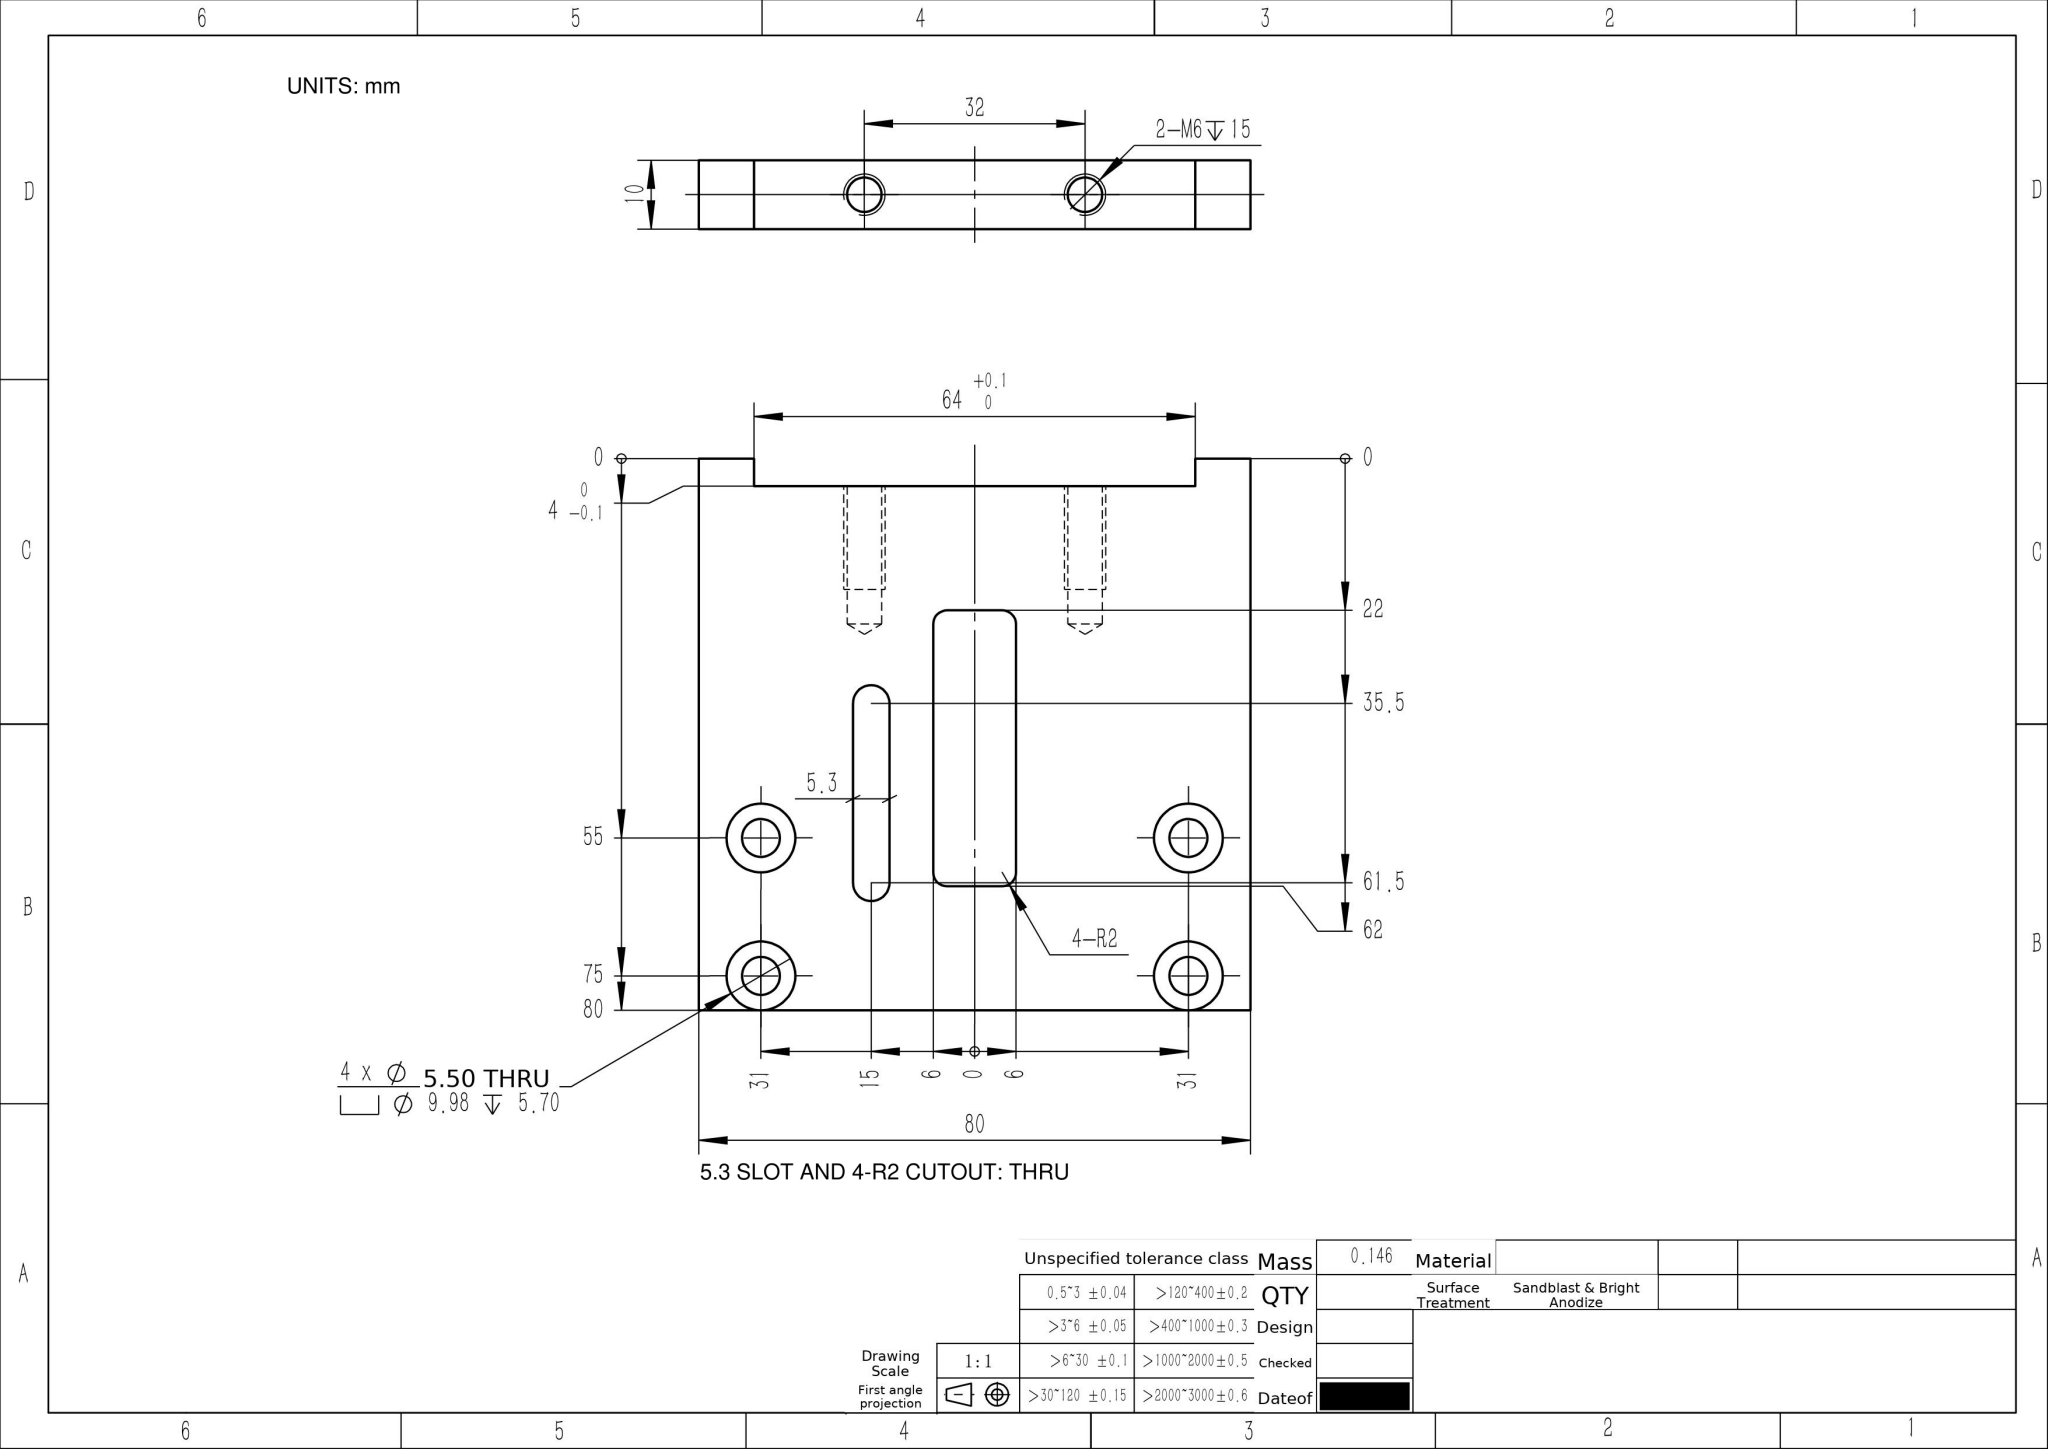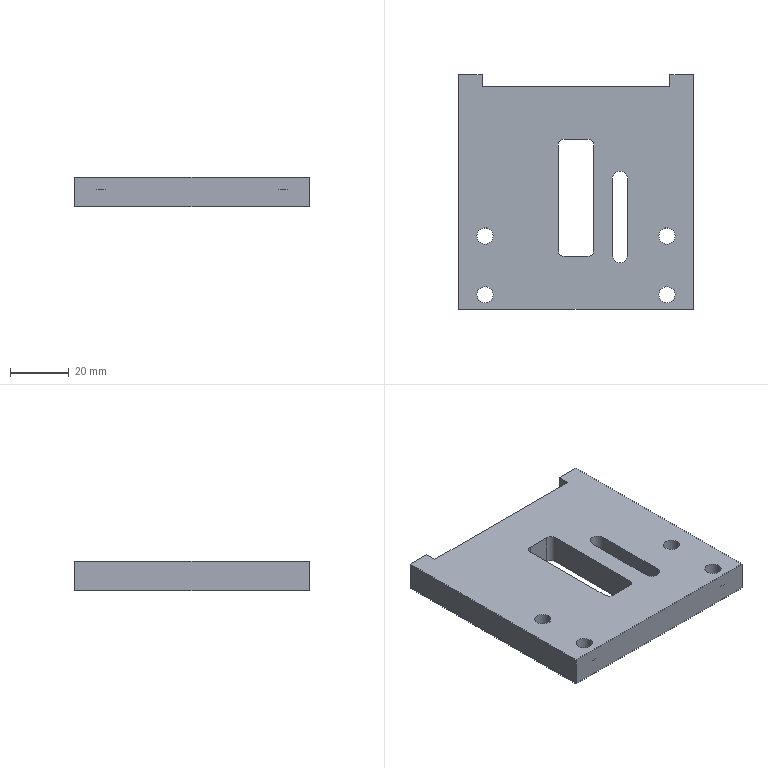Part | NX | mm | 1 solid | 50 faces | box 80 x 80 x 10 mm | volume 52078 mm3 | cylinder 26 | plane 20 | cone 4 | commonest cylinder face diameters 9.98 x8 5.5 x8 5 x4 4 x4 5.3 x2